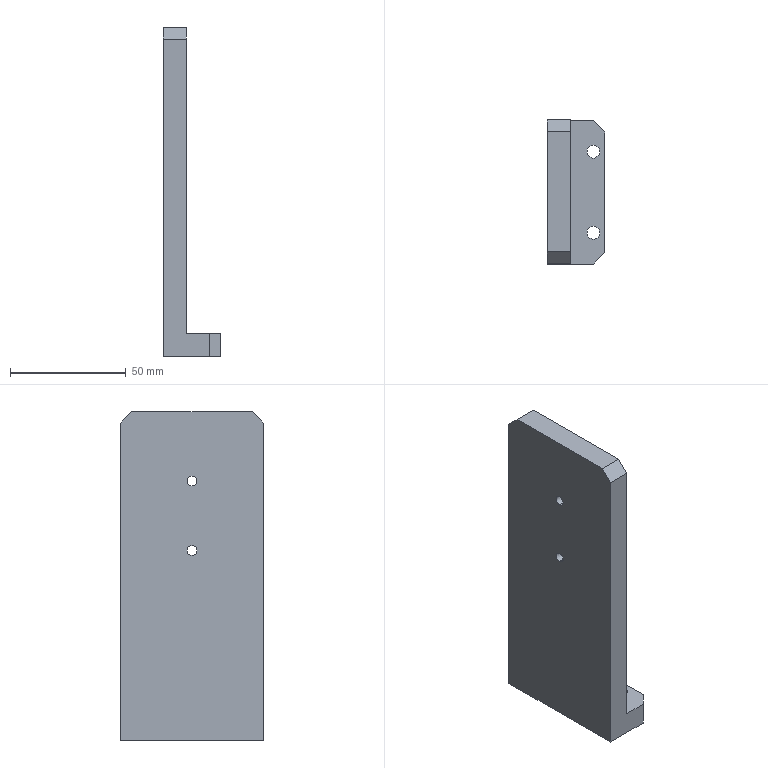Component | SolidWorks | P-SLJ-005-3_P-SLJ-005-001-1 | 1 solid | 20 faces | box 25 x 62 x 142 mm | volume 96088 mm3 | plane 12 | cylinder 8 | commonest cylinder face diameters 4.2 x4 5.5 x4 | material A3
build123d program:
from build123d import *

# Parameters (mm, degrees)
EXTRUDE1_DEPTH       = 31
M5_CLEARANCE_HOLE1_D = 5.5
M5_TAPPED_HOLE1_D    = 4.2
CHAMFER1_SIZE        = 5
CHAMFER2_SIZE        = 5


with BuildPart() as part:
    # Sketch1 → Extrude1 (new, symmetric)
    with BuildSketch(Plane(origin=(0, 0, 0), x_dir=(1, 0, 0), z_dir=(0, 1, 0))):
        Polygon((0, 0), (142, 0), (142, -10), (10, -10), (10, -25), (0, -25), align=None)
    extrude(amount=EXTRUDE1_DEPTH, both=True)

    # M5 Clearance Hole1 (through all)
    with Locations(Plane(origin=(10, 0, 0), x_dir=(0, 0, -1), z_dir=(1, 0, 0))):
        with Locations((-20, 17.5), (-20, -17.5)):
            Hole(M5_CLEARANCE_HOLE1_D / 2)

    # M5 Tapped Hole1 (through all)
    with Locations(Plane(origin=(0, 0, 0), x_dir=(-1, 0, 0), z_dir=(0, 0, -1))):
        with Locations((-112, 0), (-82, 0)):
            Hole(M5_TAPPED_HOLE1_D / 2)

    # Chamfer1
    chamfer1_edges = [part.edges().sort_by_distance(p)[0] for p in [
        (142, 31, 5),
        (142, -31, 5),
    ]]
    chamfer(chamfer1_edges, length=CHAMFER1_SIZE)

    # Chamfer2
    chamfer2_edges = [part.edges().sort_by_distance(p)[0] for p in [
        (5, 31, 25),
        (5, -31, 25),
    ]]
    chamfer(chamfer2_edges, length=CHAMFER2_SIZE)


solid = part.part

# Placed as in the assembly
solid = solid.moved(Location((-49.5, 15.5, 1235.634), (180, 90, 0)))
STEP:
#1=COLOUR_RGB('',0.7922,0.8196,0.9333);
#2=FILL_AREA_STYLE_COLOUR('',#1);
#3=FILL_AREA_STYLE('',(#2));
#4=SURFACE_STYLE_FILL_AREA(#3);
#5=SURFACE_SIDE_STYLE('',(#4));
#6=SURFACE_STYLE_USAGE(.BOTH.,#5);
#7=PRESENTATION_STYLE_ASSIGNMENT((#6));
#8=CARTESIAN_POINT('',(-1.555,0.6102,53.139));
#9=VERTEX_POINT('',#8);
#10=CARTESIAN_POINT('',(-1.555,0.6102,52.974));
#11=VERTEX_POINT('',#10);
#12=CARTESIAN_POINT('',(-1.555,0.6102,53.056));
#13=DIRECTION('',(-1.,-0.,-0.));
#14=DIRECTION('',(0.,0.,-1.));
#15=AXIS2_PLACEMENT_3D('',#12,#13,#14);
#16=CIRCLE('',#15,0.08268);
#17=EDGE_CURVE('',#9,#11,#16,.T.);
#18=ORIENTED_EDGE('',*,*,#17,.F.);
#19=CARTESIAN_POINT('',(-1.949,0.6102,53.139));
#20=VERTEX_POINT('',#19);
#21=CARTESIAN_POINT('',(-1.949,0.6102,53.139));
#22=DIRECTION('',(-1.,-0.,-0.));
#23=VECTOR('',#22,39.37);
#24=LINE('',#21,#23);
#25=EDGE_CURVE('',#9,#20,#24,.T.);
#26=ORIENTED_EDGE('',*,*,#25,.T.);
#27=CARTESIAN_POINT('',(-1.949,0.6102,52.974));
#28=VERTEX_POINT('',#27);
#29=CARTESIAN_POINT('',(-1.949,0.6102,53.056));
#30=DIRECTION('',(-1.,-0.,-0.));
#31=DIRECTION('',(0.,0.,-1.));
#32=AXIS2_PLACEMENT_3D('',#29,#30,#31);
#33=CIRCLE('',#32,0.08268);
#34=EDGE_CURVE('',#20,#28,#33,.T.);
#35=ORIENTED_EDGE('',*,*,#34,.T.);
#36=CARTESIAN_POINT('',(-1.949,0.6102,52.974));
#37=DIRECTION('',(-1.,-0.,-0.));
#38=VECTOR('',#37,39.37);
#39=LINE('',#36,#38);
#40=EDGE_CURVE('',#11,#28,#39,.T.);
#41=ORIENTED_EDGE('',*,*,#40,.F.);
#42=EDGE_LOOP('',(#18,#26,#35,#41));
#43=FACE_OUTER_BOUND('',#42,.T.);
#44=CARTESIAN_POINT('',(-1.949,0.6102,53.056));
#45=DIRECTION('',(-1.,-0.,-0.));
#46=DIRECTION('',(0.,0.,-1.));
#47=AXIS2_PLACEMENT_3D('',#44,#45,#46);
#48=CYLINDRICAL_SURFACE('',#47,0.08268);
#49=ADVANCED_FACE('',(#43),#48,.F.);
#50=CARTESIAN_POINT('',(-1.555,0.6102,51.958));
#51=VERTEX_POINT('',#50);
#52=CARTESIAN_POINT('',(-1.555,0.6102,51.793));
#53=VERTEX_POINT('',#52);
#54=CARTESIAN_POINT('',(-1.555,0.6102,51.875));
#55=DIRECTION('',(-1.,-0.,-0.));
#56=DIRECTION('',(0.,0.,-1.));
#57=AXIS2_PLACEMENT_3D('',#54,#55,#56);
#58=CIRCLE('',#57,0.08268);
#59=EDGE_CURVE('',#51,#53,#58,.T.);
#60=ORIENTED_EDGE('',*,*,#59,.F.);
#61=CARTESIAN_POINT('',(-1.949,0.6102,51.958));
#62=VERTEX_POINT('',#61);
#63=CARTESIAN_POINT('',(-1.949,0.6102,51.958));
#64=DIRECTION('',(-1.,-0.,-0.));
#65=VECTOR('',#64,39.37);
#66=LINE('',#63,#65);
#67=EDGE_CURVE('',#51,#62,#66,.T.);
#68=ORIENTED_EDGE('',*,*,#67,.T.);
#69=CARTESIAN_POINT('',(-1.949,0.6102,51.793));
#70=VERTEX_POINT('',#69);
#71=CARTESIAN_POINT('',(-1.949,0.6102,51.875));
#72=DIRECTION('',(-1.,-0.,-0.));
#73=DIRECTION('',(0.,0.,-1.));
#74=AXIS2_PLACEMENT_3D('',#71,#72,#73);
#75=CIRCLE('',#74,0.08268);
#76=EDGE_CURVE('',#62,#70,#75,.T.);
#77=ORIENTED_EDGE('',*,*,#76,.T.);
#78=CARTESIAN_POINT('',(-1.949,0.6102,51.793));
#79=DIRECTION('',(-1.,-0.,-0.));
#80=VECTOR('',#79,39.37);
#81=LINE('',#78,#80);
#82=EDGE_CURVE('',#53,#70,#81,.T.);
#83=ORIENTED_EDGE('',*,*,#82,.F.);
#84=EDGE_LOOP('',(#60,#68,#77,#83));
#85=FACE_OUTER_BOUND('',#84,.T.);
#86=CARTESIAN_POINT('',(-1.949,0.6102,51.875));
#87=DIRECTION('',(-1.,-0.,-0.));
#88=DIRECTION('',(0.,0.,-1.));
#89=AXIS2_PLACEMENT_3D('',#86,#87,#88);
#90=CYLINDRICAL_SURFACE('',#89,0.08268);
#91=ADVANCED_FACE('',(#85),#90,.F.);
#92=CARTESIAN_POINT('',(-1.053,-0.07874,48.647));
#93=VERTEX_POINT('',#92);
#94=CARTESIAN_POINT('',(-1.27,-0.07874,48.647));
#95=VERTEX_POINT('',#94);
#96=CARTESIAN_POINT('',(-1.161,-0.07874,48.647));
#97=DIRECTION('',(-0.,-0.,1.));
#98=DIRECTION('',(-1.,-0.,0.));
#99=AXIS2_PLACEMENT_3D('',#96,#97,#98);
#100=CIRCLE('',#99,0.1083);
#101=EDGE_CURVE('',#93,#95,#100,.T.);
#102=ORIENTED_EDGE('',*,*,#101,.F.);
#103=CARTESIAN_POINT('',(-1.053,-0.07874,49.041));
#104=VERTEX_POINT('',#103);
#105=CARTESIAN_POINT('',(-1.053,-0.07874,49.041));
#106=DIRECTION('',(-0.,-0.,1.));
#107=VECTOR('',#106,39.37);
#108=LINE('',#105,#107);
#109=EDGE_CURVE('',#93,#104,#108,.T.);
#110=ORIENTED_EDGE('',*,*,#109,.T.);
#111=CARTESIAN_POINT('',(-1.27,-0.07874,49.041));
#112=VERTEX_POINT('',#111);
#113=CARTESIAN_POINT('',(-1.161,-0.07874,49.041));
#114=DIRECTION('',(-0.,-0.,1.));
#115=DIRECTION('',(-1.,-0.,0.));
#116=AXIS2_PLACEMENT_3D('',#113,#114,#115);
#117=CIRCLE('',#116,0.1083);
#118=EDGE_CURVE('',#104,#112,#117,.T.);
#119=ORIENTED_EDGE('',*,*,#118,.T.);
#120=CARTESIAN_POINT('',(-1.27,-0.07874,49.041));
#121=DIRECTION('',(-0.,-0.,1.));
#122=VECTOR('',#121,39.37);
#123=LINE('',#120,#122);
#124=EDGE_CURVE('',#95,#112,#123,.T.);
#125=ORIENTED_EDGE('',*,*,#124,.F.);
#126=EDGE_LOOP('',(#102,#110,#119,#125));
#127=FACE_OUTER_BOUND('',#126,.T.);
#128=CARTESIAN_POINT('',(-1.161,-0.07874,49.041));
#129=DIRECTION('',(-0.,-0.,1.));
#130=DIRECTION('',(-1.,-0.,0.));
#131=AXIS2_PLACEMENT_3D('',#128,#129,#130);
#132=CYLINDRICAL_SURFACE('',#131,0.1083);
#133=ADVANCED_FACE('',(#127),#132,.F.);
#134=CARTESIAN_POINT('',(-1.053,1.299,48.647));
#135=VERTEX_POINT('',#134);
#136=CARTESIAN_POINT('',(-1.27,1.299,48.647));
#137=VERTEX_POINT('',#136);
#138=CARTESIAN_POINT('',(-1.161,1.299,48.647));
#139=DIRECTION('',(-0.,-0.,1.));
#140=DIRECTION('',(-1.,0.,0.));
#141=AXIS2_PLACEMENT_3D('',#138,#139,#140);
#142=CIRCLE('',#141,0.1083);
#143=EDGE_CURVE('',#135,#137,#142,.T.);
#144=ORIENTED_EDGE('',*,*,#143,.F.);
#145=CARTESIAN_POINT('',(-1.053,1.299,49.041));
#146=VERTEX_POINT('',#145);
#147=CARTESIAN_POINT('',(-1.053,1.299,49.041));
#148=DIRECTION('',(-0.,-0.,1.));
#149=VECTOR('',#148,39.37);
#150=LINE('',#147,#149);
#151=EDGE_CURVE('',#135,#146,#150,.T.);
#152=ORIENTED_EDGE('',*,*,#151,.T.);
#153=CARTESIAN_POINT('',(-1.27,1.299,49.041));
#154=VERTEX_POINT('',#153);
#155=CARTESIAN_POINT('',(-1.161,1.299,49.041));
#156=DIRECTION('',(-0.,-0.,1.));
#157=DIRECTION('',(-1.,0.,0.));
#158=AXIS2_PLACEMENT_3D('',#155,#156,#157);
#159=CIRCLE('',#158,0.1083);
#160=EDGE_CURVE('',#146,#154,#159,.T.);
#161=ORIENTED_EDGE('',*,*,#160,.T.);
#162=CARTESIAN_POINT('',(-1.27,1.299,49.041));
#163=DIRECTION('',(-0.,-0.,1.));
#164=VECTOR('',#163,39.37);
#165=LINE('',#162,#164);
#166=EDGE_CURVE('',#137,#154,#165,.T.);
#167=ORIENTED_EDGE('',*,*,#166,.F.);
#168=EDGE_LOOP('',(#144,#152,#161,#167));
#169=FACE_OUTER_BOUND('',#168,.T.);
#170=CARTESIAN_POINT('',(-1.161,1.299,49.041));
#171=DIRECTION('',(-0.,-0.,1.));
#172=DIRECTION('',(-1.,0.,0.));
#173=AXIS2_PLACEMENT_3D('',#170,#171,#172);
#174=CYLINDRICAL_SURFACE('',#173,0.1083);
#175=ADVANCED_FACE('',(#169),#174,.F.);
#176=CARTESIAN_POINT('',(-1.161,-0.07874,49.041));
#177=DIRECTION('',(-0.,-0.,1.));
#178=DIRECTION('',(-1.,-0.,0.));
#179=AXIS2_PLACEMENT_3D('',#176,#177,#178);
#180=CIRCLE('',#179,0.1083);
#181=EDGE_CURVE('',#112,#104,#180,.T.);
#182=ORIENTED_EDGE('',*,*,#181,.F.);
#183=ORIENTED_EDGE('',*,*,#118,.F.);
#184=EDGE_LOOP('',(#182,#183));
#185=FACE_BOUND('',#184,.T.);
#186=CARTESIAN_POINT('',(-0.9646,-0.4134,49.041));
#187=VERTEX_POINT('',#186);
#188=CARTESIAN_POINT('',(-0.9646,1.634,49.041));
#189=VERTEX_POINT('',#188);
#190=CARTESIAN_POINT('',(-0.9646,-0.6102,49.041));
#191=DIRECTION('',(-0.,1.,0.));
#192=VECTOR('',#191,39.37);
#193=LINE('',#190,#192);
#194=EDGE_CURVE('',#187,#189,#193,.T.);
#195=ORIENTED_EDGE('',*,*,#194,.T.);
#196=CARTESIAN_POINT('',(-1.161,1.831,49.041));
#197=VERTEX_POINT('',#196);
#198=CARTESIAN_POINT('',(-0.9646,1.634,49.041));
#199=DIRECTION('',(-0.7071,0.7071,0.));
#200=VECTOR('',#199,39.37);
#201=LINE('',#198,#200);
#202=EDGE_CURVE('',#189,#197,#201,.T.);
#203=ORIENTED_EDGE('',*,*,#202,.T.);
#204=CARTESIAN_POINT('',(-1.555,1.831,49.041));
#205=VERTEX_POINT('',#204);
#206=CARTESIAN_POINT('',(-0.9646,1.831,49.041));
#207=DIRECTION('',(-1.,-0.,-0.));
#208=VECTOR('',#207,39.37);
#209=LINE('',#206,#208);
#210=EDGE_CURVE('',#197,#205,#209,.T.);
#211=ORIENTED_EDGE('',*,*,#210,.T.);
#212=CARTESIAN_POINT('',(-1.555,-0.6102,49.041));
#213=VERTEX_POINT('',#212);
#214=CARTESIAN_POINT('',(-1.555,-0.6102,49.041));
#215=DIRECTION('',(-0.,1.,0.));
#216=VECTOR('',#215,39.37);
#217=LINE('',#214,#216);
#218=EDGE_CURVE('',#213,#205,#217,.T.);
#219=ORIENTED_EDGE('',*,*,#218,.F.);
#220=CARTESIAN_POINT('',(-1.161,-0.6102,49.041));
#221=VERTEX_POINT('',#220);
#222=CARTESIAN_POINT('',(-0.9646,-0.6102,49.041));
#223=DIRECTION('',(-1.,-0.,-0.));
#224=VECTOR('',#223,39.37);
#225=LINE('',#222,#224);
#226=EDGE_CURVE('',#221,#213,#225,.T.);
#227=ORIENTED_EDGE('',*,*,#226,.F.);
#228=CARTESIAN_POINT('',(-1.161,-0.6102,49.041));
#229=DIRECTION('',(0.7071,0.7071,0.));
#230=VECTOR('',#229,39.37);
#231=LINE('',#228,#230);
#232=EDGE_CURVE('',#221,#187,#231,.T.);
#233=ORIENTED_EDGE('',*,*,#232,.T.);
#234=EDGE_LOOP('',(#195,#203,#211,#219,#227,#233));
#235=FACE_OUTER_BOUND('',#234,.T.);
#236=CARTESIAN_POINT('',(-1.161,1.299,49.041));
#237=DIRECTION('',(-0.,-0.,1.));
#238=DIRECTION('',(-1.,0.,0.));
#239=AXIS2_PLACEMENT_3D('',#236,#237,#238);
#240=CIRCLE('',#239,0.1083);
#241=EDGE_CURVE('',#154,#146,#240,.T.);
#242=ORIENTED_EDGE('',*,*,#241,.F.);
#243=ORIENTED_EDGE('',*,*,#160,.F.);
#244=EDGE_LOOP('',(#242,#243));
#245=FACE_BOUND('',#244,.T.);
#246=CARTESIAN_POINT('',(-0.9646,-0.6102,49.041));
#247=DIRECTION('',(0.,0.,-1.));
#248=DIRECTION('',(1.,0.,0.));
#249=AXIS2_PLACEMENT_3D('',#246,#247,#248);
#250=PLANE('',#249);
#251=ADVANCED_FACE('',(#185,#235,#245),#250,.F.);
#252=CARTESIAN_POINT('',(-1.161,-0.07874,48.647));
#253=DIRECTION('',(-0.,-0.,1.));
#254=DIRECTION('',(-1.,-0.,0.));
#255=AXIS2_PLACEMENT_3D('',#252,#253,#254);
#256=CIRCLE('',#255,0.1083);
#257=EDGE_CURVE('',#95,#93,#256,.T.);
#258=ORIENTED_EDGE('',*,*,#257,.T.);
#259=ORIENTED_EDGE('',*,*,#101,.T.);
#260=EDGE_LOOP('',(#258,#259));
#261=FACE_BOUND('',#260,.T.);
#262=CARTESIAN_POINT('',(-1.161,1.299,48.647));
#263=DIRECTION('',(-0.,-0.,1.));
#264=DIRECTION('',(-1.,0.,0.));
#265=AXIS2_PLACEMENT_3D('',#262,#263,#264);
#266=CIRCLE('',#265,0.1083);
#267=EDGE_CURVE('',#137,#135,#266,.T.);
#268=ORIENTED_EDGE('',*,*,#267,.T.);
#269=ORIENTED_EDGE('',*,*,#143,.T.);
#270=EDGE_LOOP('',(#268,#269));
#271=FACE_BOUND('',#270,.T.);
#272=CARTESIAN_POINT('',(-1.949,1.831,48.647));
#273=VERTEX_POINT('',#272);
#274=CARTESIAN_POINT('',(-1.161,1.831,48.647));
#275=VERTEX_POINT('',#274);
#276=CARTESIAN_POINT('',(-1.949,1.831,48.647));
#277=DIRECTION('',(1.,0.,0.));
#278=VECTOR('',#277,39.37);
#279=LINE('',#276,#278);
#280=EDGE_CURVE('',#273,#275,#279,.T.);
#281=ORIENTED_EDGE('',*,*,#280,.T.);
#282=CARTESIAN_POINT('',(-0.9646,1.634,48.647));
#283=VERTEX_POINT('',#282);
#284=CARTESIAN_POINT('',(-0.9646,1.634,48.647));
#285=DIRECTION('',(0.7071,-0.7071,-0.));
#286=VECTOR('',#285,39.37);
#287=LINE('',#284,#286);
#288=EDGE_CURVE('',#275,#283,#287,.T.);
#289=ORIENTED_EDGE('',*,*,#288,.T.);
#290=CARTESIAN_POINT('',(-0.9646,-0.4134,48.647));
#291=VERTEX_POINT('',#290);
#292=CARTESIAN_POINT('',(-0.9646,-0.6102,48.647));
#293=DIRECTION('',(-0.,1.,0.));
#294=VECTOR('',#293,39.37);
#295=LINE('',#292,#294);
#296=EDGE_CURVE('',#291,#283,#295,.T.);
#297=ORIENTED_EDGE('',*,*,#296,.F.);
#298=CARTESIAN_POINT('',(-1.161,-0.6102,48.647));
#299=VERTEX_POINT('',#298);
#300=CARTESIAN_POINT('',(-1.161,-0.6102,48.647));
#301=DIRECTION('',(-0.7071,-0.7071,-0.));
#302=VECTOR('',#301,39.37);
#303=LINE('',#300,#302);
#304=EDGE_CURVE('',#291,#299,#303,.T.);
#305=ORIENTED_EDGE('',*,*,#304,.T.);
#306=CARTESIAN_POINT('',(-1.949,-0.6102,48.647));
#307=VERTEX_POINT('',#306);
#308=CARTESIAN_POINT('',(-1.949,-0.6102,48.647));
#309=DIRECTION('',(1.,0.,0.));
#310=VECTOR('',#309,39.37);
#311=LINE('',#308,#310);
#312=EDGE_CURVE('',#307,#299,#311,.T.);
#313=ORIENTED_EDGE('',*,*,#312,.F.);
#314=CARTESIAN_POINT('',(-1.949,-0.6102,48.647));
#315=DIRECTION('',(-0.,1.,0.));
#316=VECTOR('',#315,39.37);
#317=LINE('',#314,#316);
#318=EDGE_CURVE('',#307,#273,#317,.T.);
#319=ORIENTED_EDGE('',*,*,#318,.T.);
#320=EDGE_LOOP('',(#281,#289,#297,#305,#313,#319));
#321=FACE_OUTER_BOUND('',#320,.T.);
#322=CARTESIAN_POINT('',(-1.949,-0.6102,48.647));
#323=DIRECTION('',(-0.,-0.,1.));
#324=DIRECTION('',(-1.,-0.,-0.));
#325=AXIS2_PLACEMENT_3D('',#322,#323,#324);
#326=PLANE('',#325);
#327=ADVANCED_FACE('',(#261,#271,#321),#326,.F.);
#328=ORIENTED_EDGE('',*,*,#296,.T.);
#329=CARTESIAN_POINT('',(-0.9646,1.634,48.647));
#330=DIRECTION('',(-0.,-0.,1.));
#331=VECTOR('',#330,39.37);
#332=LINE('',#329,#331);
#333=EDGE_CURVE('',#283,#189,#332,.T.);
#334=ORIENTED_EDGE('',*,*,#333,.T.);
#335=ORIENTED_EDGE('',*,*,#194,.F.);
#336=CARTESIAN_POINT('',(-0.9646,-0.4134,48.647));
#337=DIRECTION('',(0.,0.,-1.));
#338=VECTOR('',#337,39.37);
#339=LINE('',#336,#338);
#340=EDGE_CURVE('',#187,#291,#339,.T.);
#341=ORIENTED_EDGE('',*,*,#340,.T.);
#342=EDGE_LOOP('',(#328,#334,#335,#341));
#343=FACE_OUTER_BOUND('',#342,.T.);
#344=CARTESIAN_POINT('',(-0.9646,-0.6102,48.647));
#345=DIRECTION('',(-1.,-0.,-0.));
#346=DIRECTION('',(0.,0.,-1.));
#347=AXIS2_PLACEMENT_3D('',#344,#345,#346);
#348=PLANE('',#347);
#349=ADVANCED_FACE('',(#343),#348,.F.);
#350=CARTESIAN_POINT('',(-1.555,0.6102,53.056));
#351=DIRECTION('',(-1.,-0.,-0.));
#352=DIRECTION('',(0.,0.,-1.));
#353=AXIS2_PLACEMENT_3D('',#350,#351,#352);
#354=CIRCLE('',#353,0.08268);
#355=EDGE_CURVE('',#11,#9,#354,.T.);
#356=ORIENTED_EDGE('',*,*,#355,.T.);
#357=ORIENTED_EDGE('',*,*,#17,.T.);
#358=EDGE_LOOP('',(#356,#357));
#359=FACE_BOUND('',#358,.T.);
#360=CARTESIAN_POINT('',(-1.555,0.6102,51.875));
#361=DIRECTION('',(-1.,-0.,-0.));
#362=DIRECTION('',(0.,0.,-1.));
#363=AXIS2_PLACEMENT_3D('',#360,#361,#362);
#364=CIRCLE('',#363,0.08268);
#365=EDGE_CURVE('',#53,#51,#364,.T.);
#366=ORIENTED_EDGE('',*,*,#365,.T.);
#367=ORIENTED_EDGE('',*,*,#59,.T.);
#368=EDGE_LOOP('',(#366,#367));
#369=FACE_BOUND('',#368,.T.);
#370=CARTESIAN_POINT('',(-1.555,1.831,54.041));
#371=VERTEX_POINT('',#370);
#372=CARTESIAN_POINT('',(-1.555,1.831,54.238));
#373=DIRECTION('',(-0.,-0.,1.));
#374=VECTOR('',#373,39.37);
#375=LINE('',#372,#374);
#376=EDGE_CURVE('',#205,#371,#375,.T.);
#377=ORIENTED_EDGE('',*,*,#376,.T.);
#378=CARTESIAN_POINT('',(-1.555,1.634,54.238));
#379=VERTEX_POINT('',#378);
#380=CARTESIAN_POINT('',(-1.555,1.634,54.238));
#381=DIRECTION('',(0.,-0.7071,0.7071));
#382=VECTOR('',#381,39.37);
#383=LINE('',#380,#382);
#384=EDGE_CURVE('',#371,#379,#383,.T.);
#385=ORIENTED_EDGE('',*,*,#384,.T.);
#386=CARTESIAN_POINT('',(-1.555,-0.4134,54.238));
#387=VERTEX_POINT('',#386);
#388=CARTESIAN_POINT('',(-1.555,-0.6102,54.238));
#389=DIRECTION('',(-0.,1.,0.));
#390=VECTOR('',#389,39.37);
#391=LINE('',#388,#390);
#392=EDGE_CURVE('',#387,#379,#391,.T.);
#393=ORIENTED_EDGE('',*,*,#392,.F.);
#394=CARTESIAN_POINT('',(-1.555,-0.6102,54.041));
#395=VERTEX_POINT('',#394);
#396=CARTESIAN_POINT('',(-1.555,-0.6102,54.041));
#397=DIRECTION('',(0.,-0.7071,-0.7071));
#398=VECTOR('',#397,39.37);
#399=LINE('',#396,#398);
#400=EDGE_CURVE('',#387,#395,#399,.T.);
#401=ORIENTED_EDGE('',*,*,#400,.T.);
#402=CARTESIAN_POINT('',(-1.555,-0.6102,54.238));
#403=DIRECTION('',(-0.,-0.,1.));
#404=VECTOR('',#403,39.37);
#405=LINE('',#402,#404);
#406=EDGE_CURVE('',#213,#395,#405,.T.);
#407=ORIENTED_EDGE('',*,*,#406,.F.);
#408=ORIENTED_EDGE('',*,*,#218,.T.);
#409=EDGE_LOOP('',(#377,#385,#393,#401,#407,#408));
#410=FACE_OUTER_BOUND('',#409,.T.);
#411=CARTESIAN_POINT('',(-1.555,-0.6102,54.238));
#412=DIRECTION('',(-1.,-0.,-0.));
#413=DIRECTION('',(0.,0.,-1.));
#414=AXIS2_PLACEMENT_3D('',#411,#412,#413);
#415=PLANE('',#414);
#416=ADVANCED_FACE('',(#359,#369,#410),#415,.F.);
#417=ORIENTED_EDGE('',*,*,#392,.T.);
#418=CARTESIAN_POINT('',(-1.949,1.634,54.238));
#419=VERTEX_POINT('',#418);
#420=CARTESIAN_POINT('',(-1.949,1.634,54.238));
#421=DIRECTION('',(-1.,-0.,-0.));
#422=VECTOR('',#421,39.37);
#423=LINE('',#420,#422);
#424=EDGE_CURVE('',#379,#419,#423,.T.);
#425=ORIENTED_EDGE('',*,*,#424,.T.);
#426=CARTESIAN_POINT('',(-1.949,-0.4134,54.238));
#427=VERTEX_POINT('',#426);
#428=CARTESIAN_POINT('',(-1.949,-0.6102,54.238));
#429=DIRECTION('',(-0.,1.,0.));
#430=VECTOR('',#429,39.37);
#431=LINE('',#428,#430);
#432=EDGE_CURVE('',#427,#419,#431,.T.);
#433=ORIENTED_EDGE('',*,*,#432,.F.);
#434=CARTESIAN_POINT('',(-1.555,-0.4134,54.238));
#435=DIRECTION('',(1.,0.,0.));
#436=VECTOR('',#435,39.37);
#437=LINE('',#434,#436);
#438=EDGE_CURVE('',#427,#387,#437,.T.);
#439=ORIENTED_EDGE('',*,*,#438,.T.);
#440=EDGE_LOOP('',(#417,#425,#433,#439));
#441=FACE_OUTER_BOUND('',#440,.T.);
#442=CARTESIAN_POINT('',(-1.949,-0.6102,54.238));
#443=DIRECTION('',(0.,0.,-1.));
#444=DIRECTION('',(1.,0.,0.));
#445=AXIS2_PLACEMENT_3D('',#442,#443,#444);
#446=PLANE('',#445);
#447=ADVANCED_FACE('',(#441),#446,.F.);
#448=CARTESIAN_POINT('',(-1.949,0.6102,53.056));
#449=DIRECTION('',(-1.,-0.,-0.));
#450=DIRECTION('',(0.,0.,-1.));
#451=AXIS2_PLACEMENT_3D('',#448,#449,#450);
#452=CIRCLE('',#451,0.08268);
#453=EDGE_CURVE('',#28,#20,#452,.T.);
#454=ORIENTED_EDGE('',*,*,#453,.F.);
#455=ORIENTED_EDGE('',*,*,#34,.F.);
#456=EDGE_LOOP('',(#454,#455));
#457=FACE_BOUND('',#456,.T.);
#458=CARTESIAN_POINT('',(-1.949,0.6102,51.875));
#459=DIRECTION('',(-1.,-0.,-0.));
#460=DIRECTION('',(0.,0.,-1.));
#461=AXIS2_PLACEMENT_3D('',#458,#459,#460);
#462=CIRCLE('',#461,0.08268);
#463=EDGE_CURVE('',#70,#62,#462,.T.);
#464=ORIENTED_EDGE('',*,*,#463,.F.);
#465=ORIENTED_EDGE('',*,*,#76,.F.);
#466=EDGE_LOOP('',(#464,#465));
#467=FACE_BOUND('',#466,.T.);
#468=ORIENTED_EDGE('',*,*,#432,.T.);
#469=CARTESIAN_POINT('',(-1.949,1.831,54.041));
#470=VERTEX_POINT('',#469);
#471=CARTESIAN_POINT('',(-1.949,1.634,54.238));
#472=DIRECTION('',(-0.,0.7071,-0.7071));
#473=VECTOR('',#472,39.37);
#474=LINE('',#471,#473);
#475=EDGE_CURVE('',#419,#470,#474,.T.);
#476=ORIENTED_EDGE('',*,*,#475,.T.);
#477=CARTESIAN_POINT('',(-1.949,1.831,48.647));
#478=DIRECTION('',(0.,0.,-1.));
#479=VECTOR('',#478,39.37);
#480=LINE('',#477,#479);
#481=EDGE_CURVE('',#470,#273,#480,.T.);
#482=ORIENTED_EDGE('',*,*,#481,.T.);
#483=ORIENTED_EDGE('',*,*,#318,.F.);
#484=CARTESIAN_POINT('',(-1.949,-0.6102,54.041));
#485=VERTEX_POINT('',#484);
#486=CARTESIAN_POINT('',(-1.949,-0.6102,48.647));
#487=DIRECTION('',(0.,0.,-1.));
#488=VECTOR('',#487,39.37);
#489=LINE('',#486,#488);
#490=EDGE_CURVE('',#485,#307,#489,.T.);
#491=ORIENTED_EDGE('',*,*,#490,.F.);
#492=CARTESIAN_POINT('',(-1.949,-0.6102,54.041));
#493=DIRECTION('',(-0.,0.7071,0.7071));
#494=VECTOR('',#493,39.37);
#495=LINE('',#492,#494);
#496=EDGE_CURVE('',#485,#427,#495,.T.);
#497=ORIENTED_EDGE('',*,*,#496,.T.);
#498=EDGE_LOOP('',(#468,#476,#482,#483,#491,#497));
#499=FACE_OUTER_BOUND('',#498,.T.);
#500=CARTESIAN_POINT('',(-1.949,-0.6102,48.647));
#501=DIRECTION('',(1.,0.,0.));
#502=DIRECTION('',(-0.,-0.,1.));
#503=AXIS2_PLACEMENT_3D('',#500,#501,#502);
#504=PLANE('',#503);
#505=ADVANCED_FACE('',(#457,#467,#499),#504,.F.);
#506=ORIENTED_EDGE('',*,*,#312,.T.);
#507=CARTESIAN_POINT('',(-1.161,-0.6102,49.041));
#508=DIRECTION('',(-0.,-0.,1.));
#509=VECTOR('',#508,39.37);
#510=LINE('',#507,#509);
#511=EDGE_CURVE('',#299,#221,#510,.T.);
#512=ORIENTED_EDGE('',*,*,#511,.T.);
#513=ORIENTED_EDGE('',*,*,#226,.T.);
#514=ORIENTED_EDGE('',*,*,#406,.T.);
#515=CARTESIAN_POINT('',(-1.949,-0.6102,54.041));
#516=DIRECTION('',(-1.,-0.,-0.));
#517=VECTOR('',#516,39.37);
#518=LINE('',#515,#517);
#519=EDGE_CURVE('',#395,#485,#518,.T.);
#520=ORIENTED_EDGE('',*,*,#519,.T.);
#521=ORIENTED_EDGE('',*,*,#490,.T.);
#522=EDGE_LOOP('',(#506,#512,#513,#514,#520,#521));
#523=FACE_OUTER_BOUND('',#522,.T.);
#524=CARTESIAN_POINT('',(-1.949,-0.6102,48.647));
#525=DIRECTION('',(0.,-1.,-0.));
#526=DIRECTION('',(1.,0.,0.));
#527=AXIS2_PLACEMENT_3D('',#524,#525,#526);
#528=PLANE('',#527);
#529=ADVANCED_FACE('',(#523),#528,.T.);
#530=ORIENTED_EDGE('',*,*,#210,.F.);
#531=CARTESIAN_POINT('',(-1.161,1.831,48.647));
#532=DIRECTION('',(0.,0.,-1.));
#533=VECTOR('',#532,39.37);
#534=LINE('',#531,#533);
#535=EDGE_CURVE('',#197,#275,#534,.T.);
#536=ORIENTED_EDGE('',*,*,#535,.T.);
#537=ORIENTED_EDGE('',*,*,#280,.F.);
#538=ORIENTED_EDGE('',*,*,#481,.F.);
#539=CARTESIAN_POINT('',(-1.949,1.831,54.041));
#540=DIRECTION('',(1.,0.,0.));
#541=VECTOR('',#540,39.37);
#542=LINE('',#539,#541);
#543=EDGE_CURVE('',#470,#371,#542,.T.);
#544=ORIENTED_EDGE('',*,*,#543,.T.);
#545=ORIENTED_EDGE('',*,*,#376,.F.);
#546=EDGE_LOOP('',(#530,#536,#537,#538,#544,#545));
#547=FACE_OUTER_BOUND('',#546,.T.);
#548=CARTESIAN_POINT('',(-1.949,1.831,48.647));
#549=DIRECTION('',(0.,-1.,-0.));
#550=DIRECTION('',(1.,0.,0.));
#551=AXIS2_PLACEMENT_3D('',#548,#549,#550);
#552=PLANE('',#551);
#553=ADVANCED_FACE('',(#547),#552,.F.);
#554=ORIENTED_EDGE('',*,*,#151,.F.);
#555=ORIENTED_EDGE('',*,*,#267,.F.);
#556=ORIENTED_EDGE('',*,*,#166,.T.);
#557=ORIENTED_EDGE('',*,*,#241,.T.);
#558=EDGE_LOOP('',(#554,#555,#556,#557));
#559=FACE_OUTER_BOUND('',#558,.T.);
#560=CARTESIAN_POINT('',(-1.161,1.299,49.041));
#561=DIRECTION('',(-0.,-0.,1.));
#562=DIRECTION('',(-1.,0.,0.));
#563=AXIS2_PLACEMENT_3D('',#560,#561,#562);
#564=CYLINDRICAL_SURFACE('',#563,0.1083);
#565=ADVANCED_FACE('',(#559),#564,.F.);
#566=ORIENTED_EDGE('',*,*,#109,.F.);
#567=ORIENTED_EDGE('',*,*,#257,.F.);
#568=ORIENTED_EDGE('',*,*,#124,.T.);
#569=ORIENTED_EDGE('',*,*,#181,.T.);
#570=EDGE_LOOP('',(#566,#567,#568,#569));
#571=FACE_OUTER_BOUND('',#570,.T.);
#572=CARTESIAN_POINT('',(-1.161,-0.07874,49.041));
#573=DIRECTION('',(-0.,-0.,1.));
#574=DIRECTION('',(-1.,-0.,0.));
#575=AXIS2_PLACEMENT_3D('',#572,#573,#574);
#576=CYLINDRICAL_SURFACE('',#575,0.1083);
#577=ADVANCED_FACE('',(#571),#576,.F.);
#578=ORIENTED_EDGE('',*,*,#67,.F.);
#579=ORIENTED_EDGE('',*,*,#365,.F.);
#580=ORIENTED_EDGE('',*,*,#82,.T.);
#581=ORIENTED_EDGE('',*,*,#463,.T.);
#582=EDGE_LOOP('',(#578,#579,#580,#581));
#583=FACE_OUTER_BOUND('',#582,.T.);
#584=CARTESIAN_POINT('',(-1.949,0.6102,51.875));
#585=DIRECTION('',(-1.,-0.,-0.));
#586=DIRECTION('',(0.,0.,-1.));
#587=AXIS2_PLACEMENT_3D('',#584,#585,#586);
#588=CYLINDRICAL_SURFACE('',#587,0.08268);
#589=ADVANCED_FACE('',(#583),#588,.F.);
#590=ORIENTED_EDGE('',*,*,#25,.F.);
#591=ORIENTED_EDGE('',*,*,#355,.F.);
#592=ORIENTED_EDGE('',*,*,#40,.T.);
#593=ORIENTED_EDGE('',*,*,#453,.T.);
#594=EDGE_LOOP('',(#590,#591,#592,#593));
#595=FACE_OUTER_BOUND('',#594,.T.);
#596=CARTESIAN_POINT('',(-1.949,0.6102,53.056));
#597=DIRECTION('',(-1.,-0.,-0.));
#598=DIRECTION('',(0.,0.,-1.));
#599=AXIS2_PLACEMENT_3D('',#596,#597,#598);
#600=CYLINDRICAL_SURFACE('',#599,0.08268);
#601=ADVANCED_FACE('',(#595),#600,.F.);
#602=ORIENTED_EDGE('',*,*,#384,.F.);
#603=ORIENTED_EDGE('',*,*,#543,.F.);
#604=ORIENTED_EDGE('',*,*,#475,.F.);
#605=ORIENTED_EDGE('',*,*,#424,.F.);
#606=EDGE_LOOP('',(#602,#603,#604,#605));
#607=FACE_OUTER_BOUND('',#606,.T.);
#608=CARTESIAN_POINT('',(-1.949,1.634,54.238));
#609=DIRECTION('',(0.,-0.7071,-0.7071));
#610=DIRECTION('',(-1.,-0.,-0.));
#611=AXIS2_PLACEMENT_3D('',#608,#609,#610);
#612=PLANE('',#611);
#613=ADVANCED_FACE('',(#607),#612,.F.);
#614=ORIENTED_EDGE('',*,*,#400,.F.);
#615=ORIENTED_EDGE('',*,*,#438,.F.);
#616=ORIENTED_EDGE('',*,*,#496,.F.);
#617=ORIENTED_EDGE('',*,*,#519,.F.);
#618=EDGE_LOOP('',(#614,#615,#616,#617));
#619=FACE_OUTER_BOUND('',#618,.T.);
#620=CARTESIAN_POINT('',(-1.949,-0.6102,54.041));
#621=DIRECTION('',(0.,-0.7071,0.7071));
#622=DIRECTION('',(1.,0.,0.));
#623=AXIS2_PLACEMENT_3D('',#620,#621,#622);
#624=PLANE('',#623);
#625=ADVANCED_FACE('',(#619),#624,.T.);
#626=ORIENTED_EDGE('',*,*,#288,.F.);
#627=ORIENTED_EDGE('',*,*,#535,.F.);
#628=ORIENTED_EDGE('',*,*,#202,.F.);
#629=ORIENTED_EDGE('',*,*,#333,.F.);
#630=EDGE_LOOP('',(#626,#627,#628,#629));
#631=FACE_OUTER_BOUND('',#630,.T.);
#632=CARTESIAN_POINT('',(-0.9646,1.634,48.647));
#633=DIRECTION('',(-0.7071,-0.7071,-0.));
#634=DIRECTION('',(-0.,-0.,1.));
#635=AXIS2_PLACEMENT_3D('',#632,#633,#634);
#636=PLANE('',#635);
#637=ADVANCED_FACE('',(#631),#636,.F.);
#638=ORIENTED_EDGE('',*,*,#304,.F.);
#639=ORIENTED_EDGE('',*,*,#340,.F.);
#640=ORIENTED_EDGE('',*,*,#232,.F.);
#641=ORIENTED_EDGE('',*,*,#511,.F.);
#642=EDGE_LOOP('',(#638,#639,#640,#641));
#643=FACE_OUTER_BOUND('',#642,.T.);
#644=CARTESIAN_POINT('',(-1.161,-0.6102,48.647));
#645=DIRECTION('',(0.7071,-0.7071,-0.));
#646=DIRECTION('',(0.,0.,-1.));
#647=AXIS2_PLACEMENT_3D('',#644,#645,#646);
#648=PLANE('',#647);
#649=ADVANCED_FACE('',(#643),#648,.T.);
#650=CLOSED_SHELL('',(#49,#91,#133,#175,#251,#327,#349,#416,#447,#505,#529,#553,#565,#577,#589,#601,#613,#625,#637,#649));
#651=MANIFOLD_SOLID_BREP('',#650);
#652=STYLED_ITEM('',(#7),#651);
#653=PRESENTATION_LAYER_ASSIGNMENT('','',(#652));
#654=CARTESIAN_POINT('',(0.,0.,0.));
#655=DIRECTION('',(0.,0.,1.));
#656=DIRECTION('',(1.,0.,0.));
#657=AXIS2_PLACEMENT_3D('',#654,#655,#656);
#658=(LENGTH_UNIT()NAMED_UNIT(*)SI_UNIT($,.METRE.));
#659=LENGTH_MEASURE_WITH_UNIT(LENGTH_MEASURE(0.0254),#658);
#660=DIMENSIONAL_EXPONENTS(1.,0.,0.,0.,0.,0.,0.);
#661=(CONVERSION_BASED_UNIT('',#659)LENGTH_UNIT()NAMED_UNIT(#660));
#662=UNCERTAINTY_MEASURE_WITH_UNIT(LENGTH_MEASURE(0.00001),#661,'','');
#663=(NAMED_UNIT(*)PLANE_ANGLE_UNIT()SI_UNIT($,.RADIAN.));
#664=(NAMED_UNIT(*)SI_UNIT($,.STERADIAN.)SOLID_ANGLE_UNIT());
#665=(GEOMETRIC_REPRESENTATION_CONTEXT(3)GLOBAL_UNCERTAINTY_ASSIGNED_CONTEXT((#662))GLOBAL_UNIT_ASSIGNED_CONTEXT((#661,#663,#664))REPRESENTATION_CONTEXT('',''));
#666=ADVANCED_BREP_SHAPE_REPRESENTATION('',(#651,#657),#665);
#667=(LENGTH_UNIT()NAMED_UNIT(*)SI_UNIT($,.METRE.));
#668=LENGTH_MEASURE_WITH_UNIT(LENGTH_MEASURE(0.0254),#667);
#669=DIMENSIONAL_EXPONENTS(1.,0.,0.,0.,0.,0.,0.);
#670=(CONVERSION_BASED_UNIT('',#668)LENGTH_UNIT()NAMED_UNIT(#669));
#671=UNCERTAINTY_MEASURE_WITH_UNIT(LENGTH_MEASURE(0.00001),#670,'','');
#672=(NAMED_UNIT(*)PLANE_ANGLE_UNIT()SI_UNIT($,.RADIAN.));
#673=(NAMED_UNIT(*)SI_UNIT($,.STERADIAN.)SOLID_ANGLE_UNIT());
#674=(GEOMETRIC_REPRESENTATION_CONTEXT(3)GLOBAL_UNCERTAINTY_ASSIGNED_CONTEXT((#671))GLOBAL_UNIT_ASSIGNED_CONTEXT((#670,#672,#673))REPRESENTATION_CONTEXT('',''));
#675=MECHANICAL_DESIGN_GEOMETRIC_PRESENTATION_REPRESENTATION('',(#652),#674);